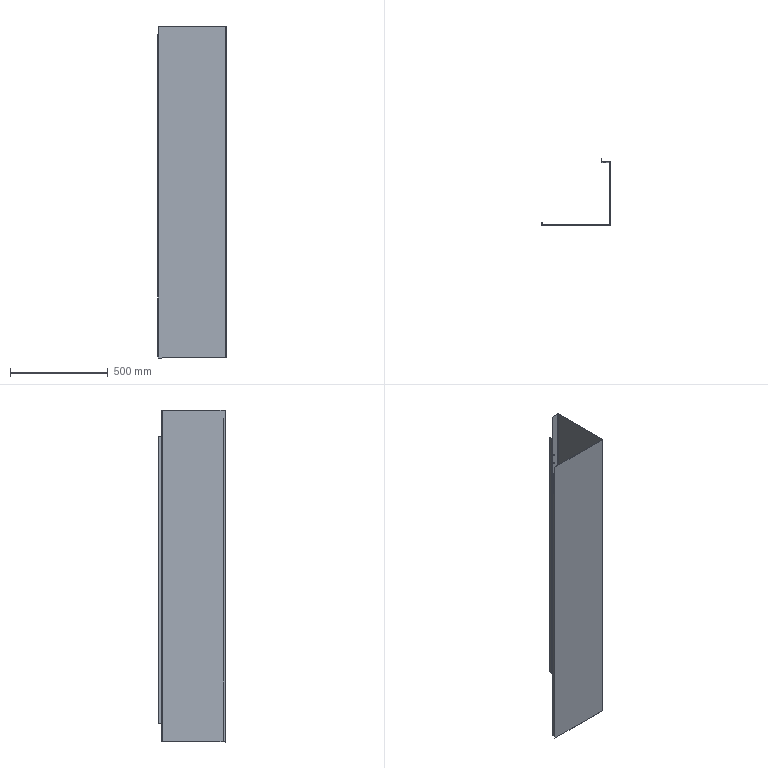Component | SolidWorks | RightSidePanel-1 | 1 solid | 61 faces | volume 1886432 mm3 | plane 41 | cylinder 20 | commonest cylinder face diameters 6.5 x12 1 x4 4 x4